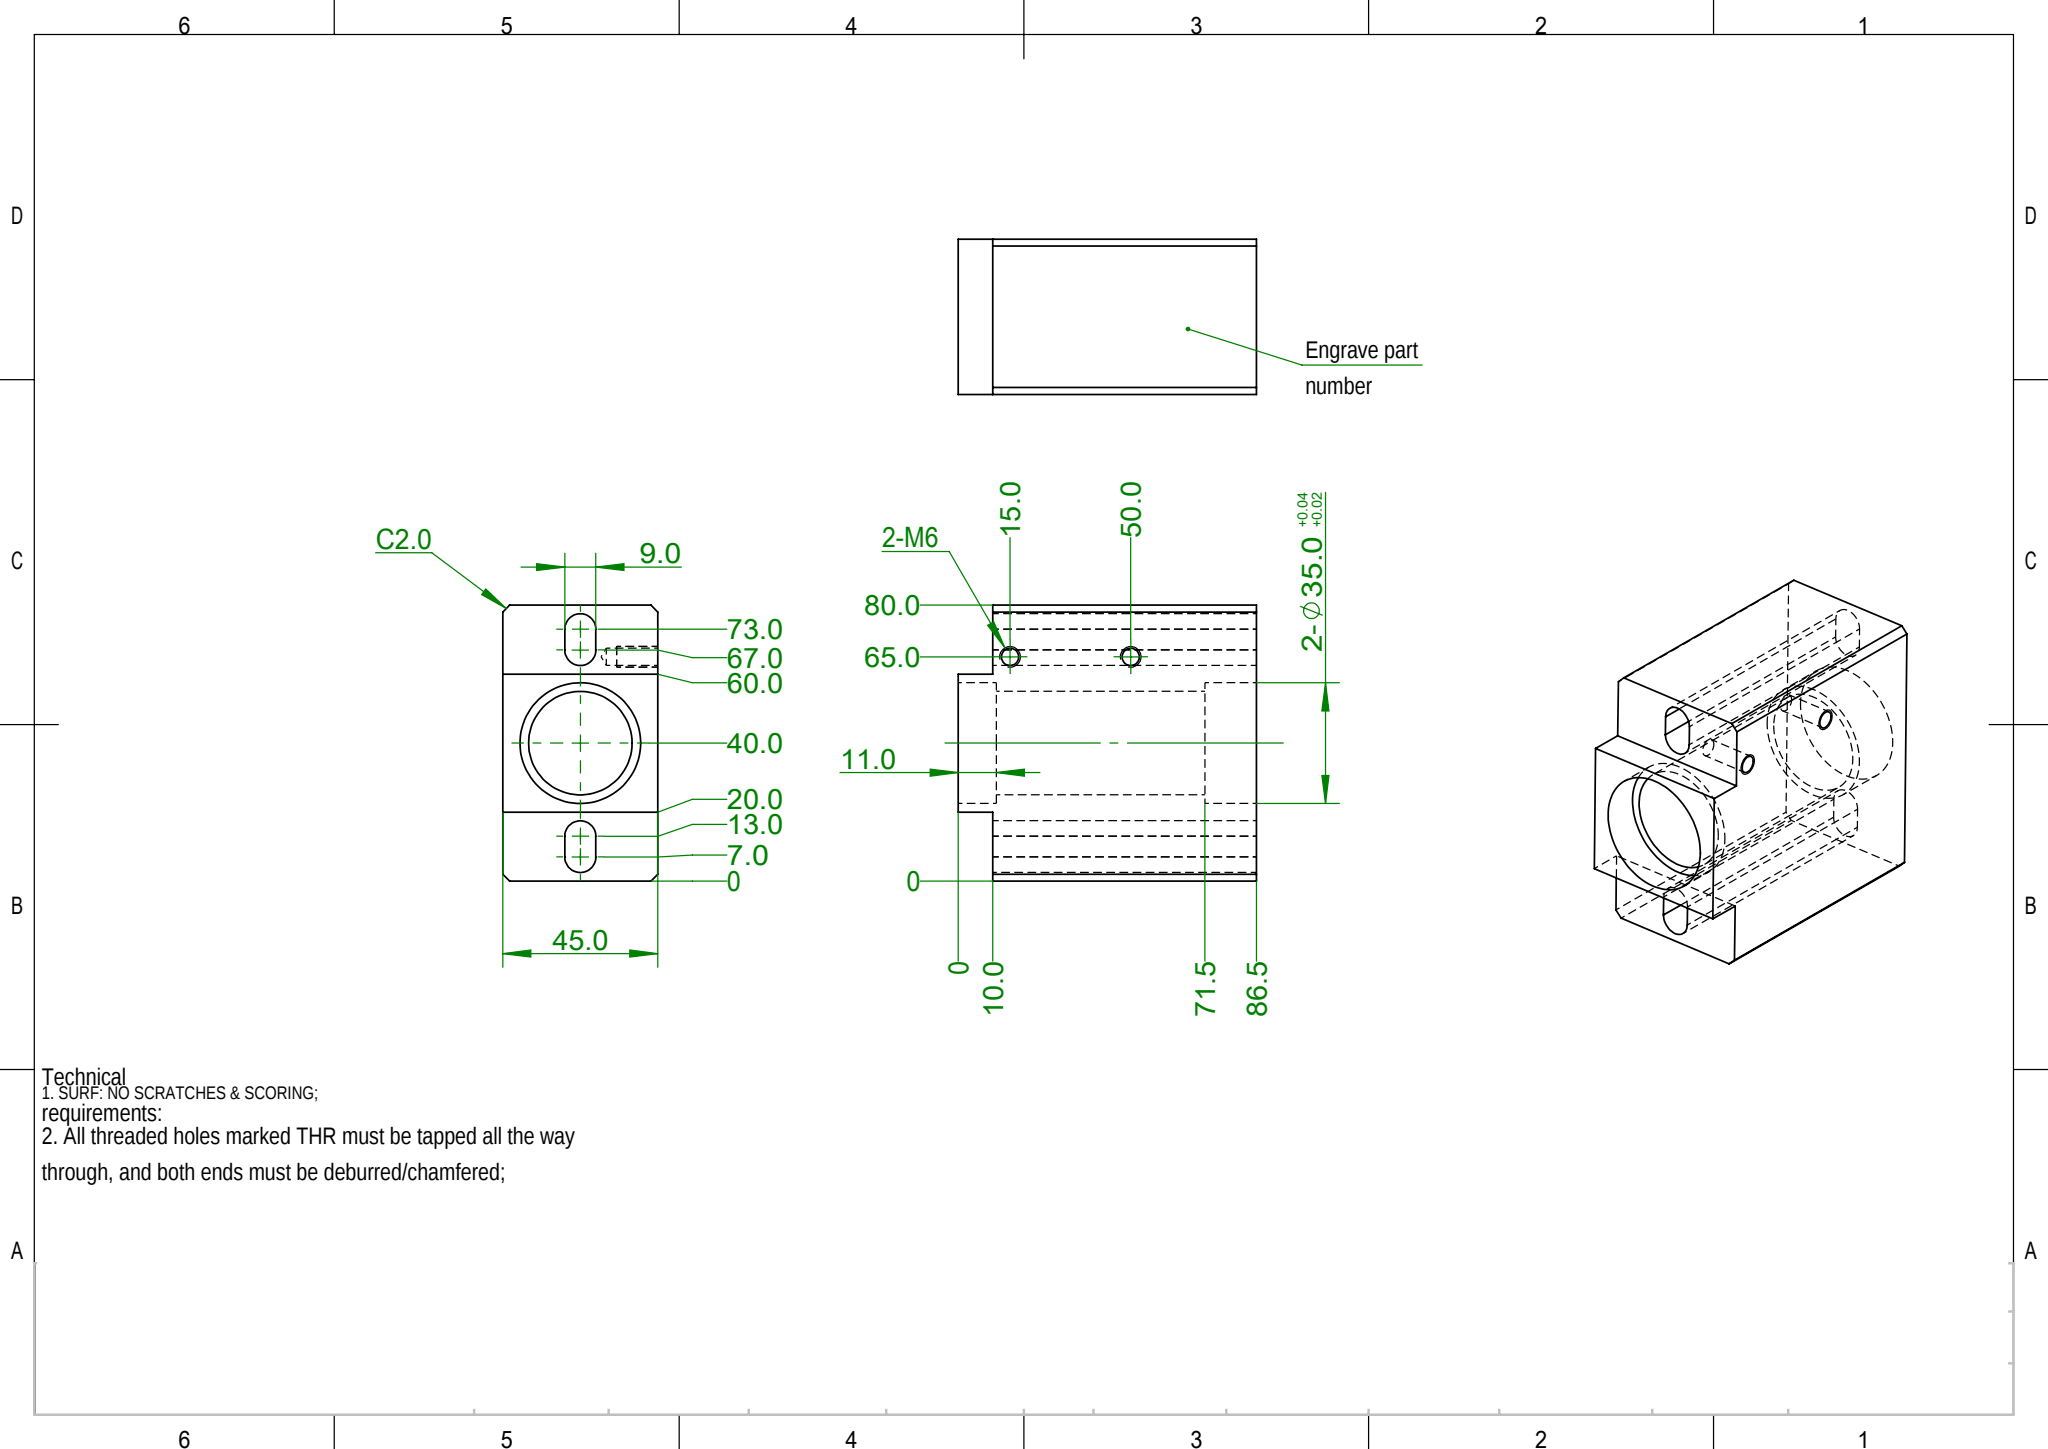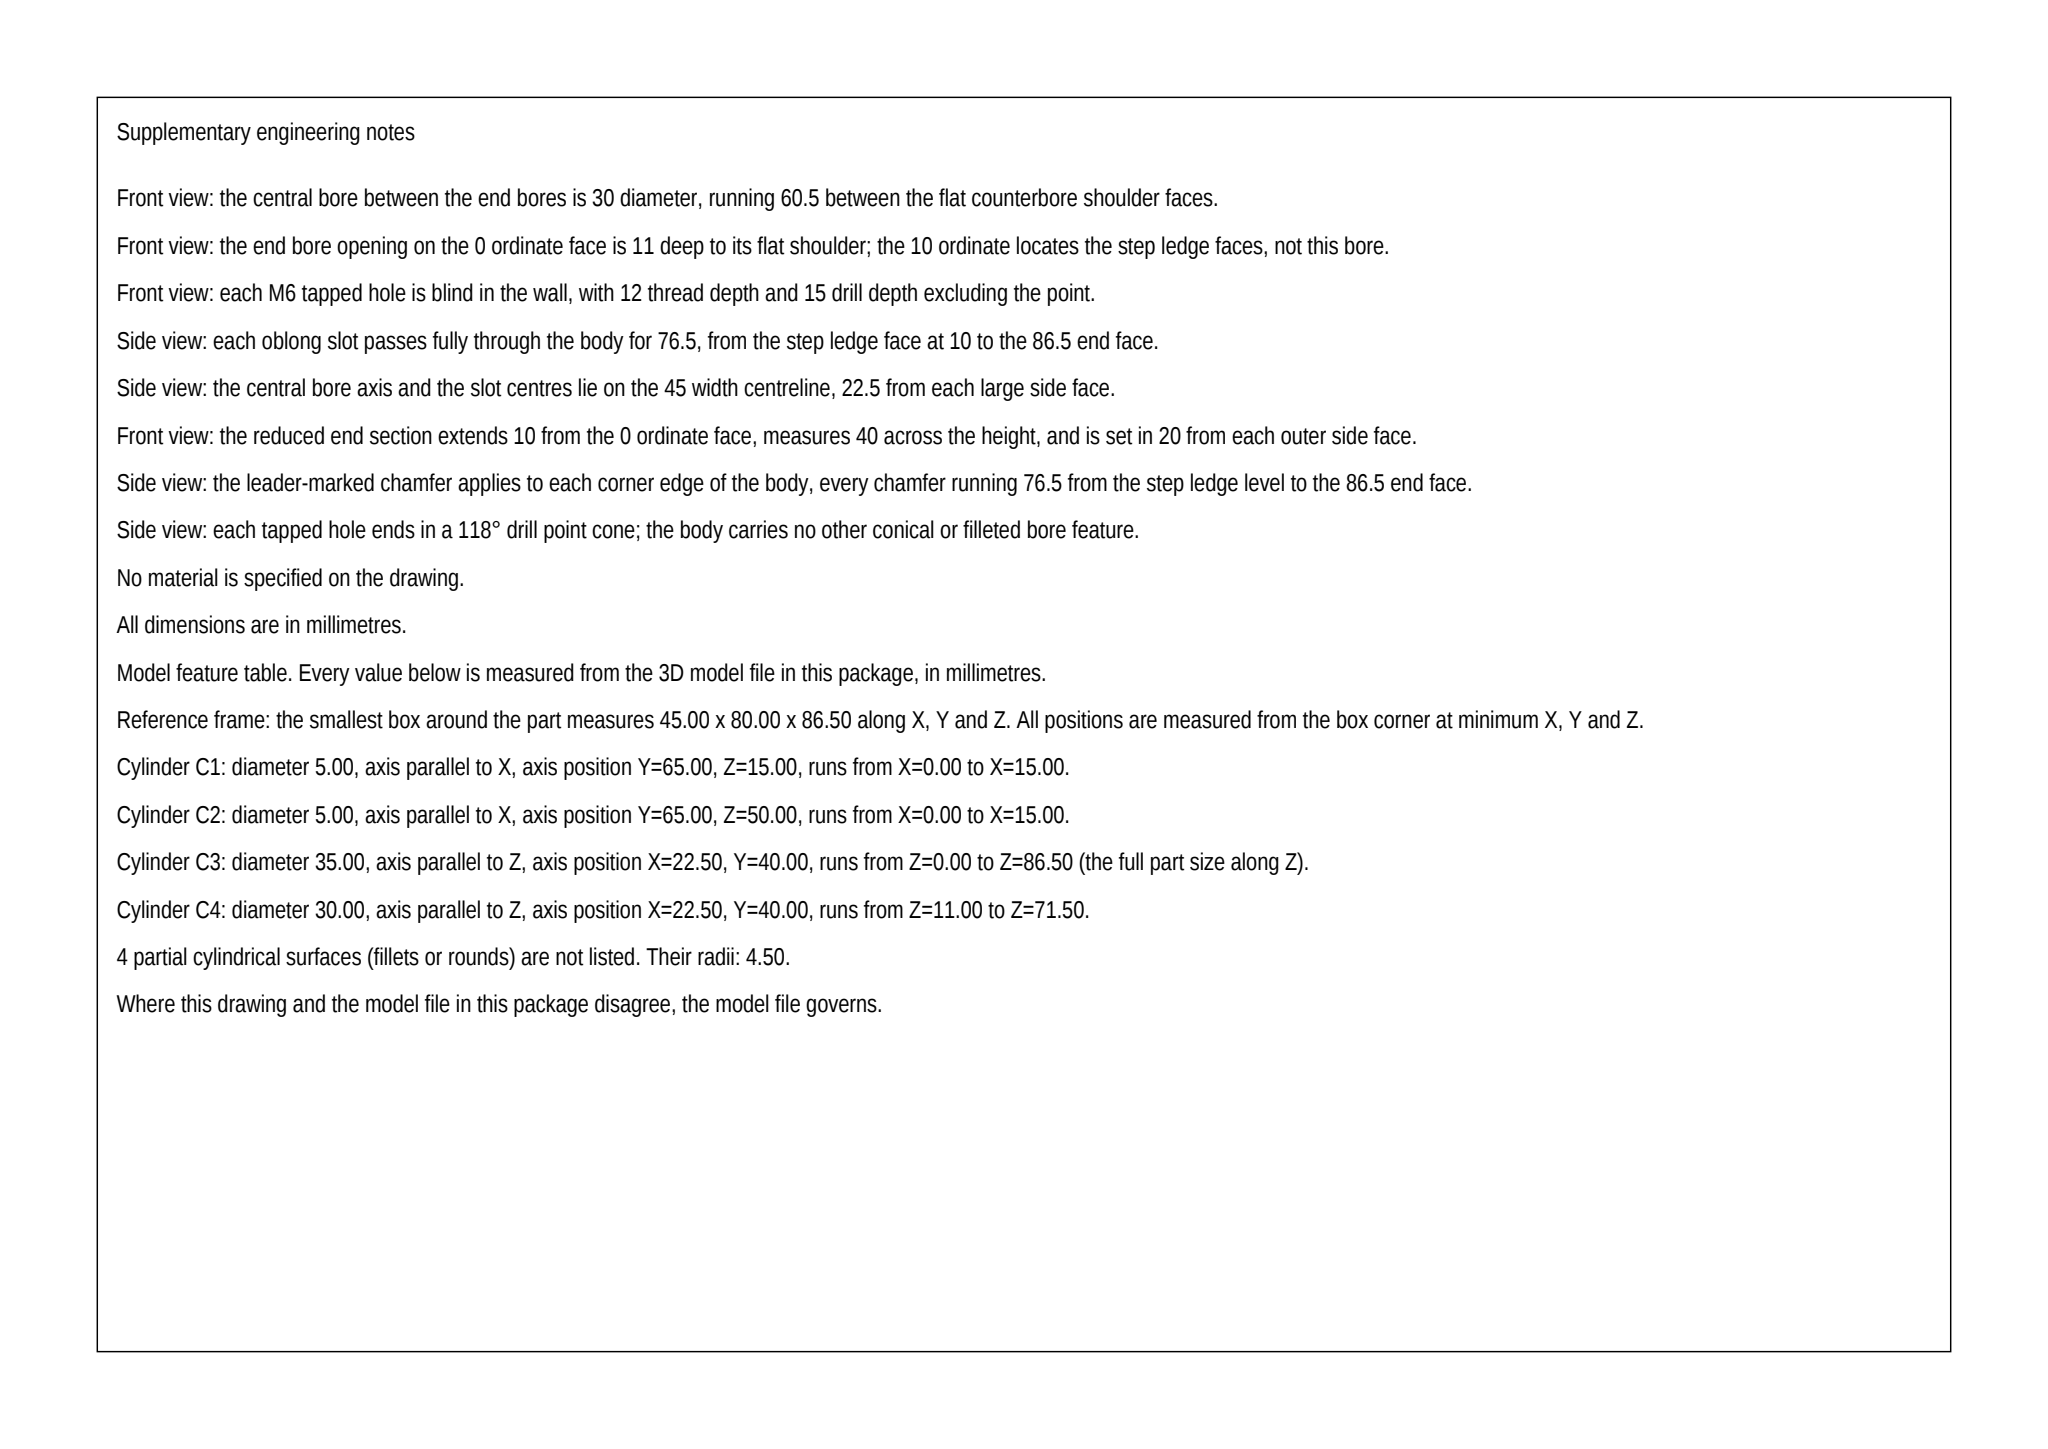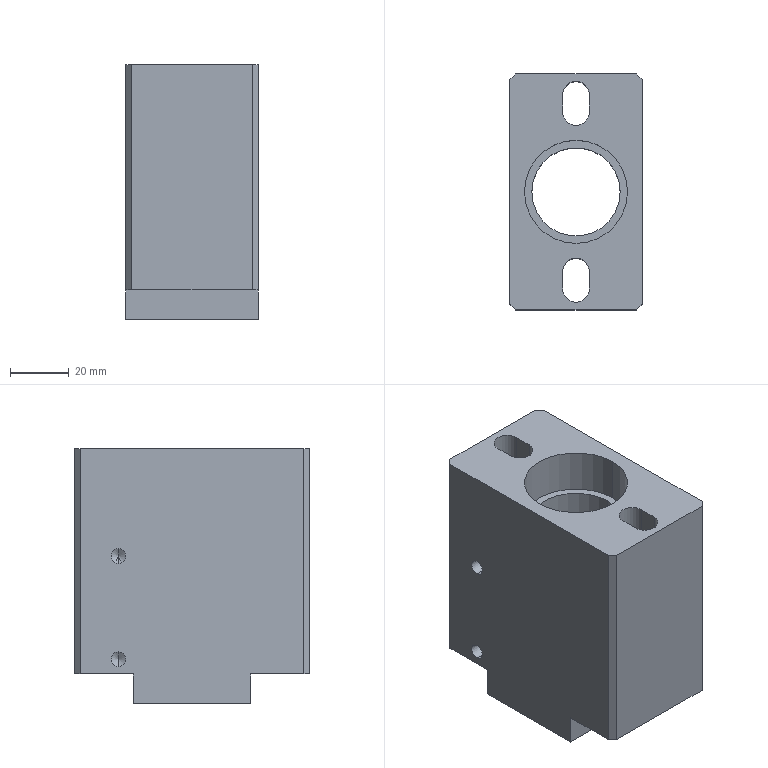Part | SolidWorks | mm | 1 solid | 38 faces | box 45 x 80 x 86.5 mm | volume 206404 mm3 | plane 20 | cylinder 14 | cone 4 | commonest cylinder face diameters 5 x4 35 x4 9 x4 30 x2
Drawing notes:
Ø30 THRU BORE BTWN 2-Ø35 C'BORES | from the solid: cyl dia 30 axis z at (22.5,40) len 60.5 between Ø35 c'bores 11 & 15 deep; 11+60.5+15=86.5 total
2-M6 DP 15 FROM NEAR FACE SHOWN IN FRONT VIEW | from the solid: 2 x Ø5 cyls axis x, len 15, at y65/z15 and y65/z50, 118° drill point; block x extent 0-45
build123d program:
from build123d import *

# Parameters (mm, degrees)
SKETCH1_W             = 45
SKETCH1_H             = 80
BOSS_EXTRUDE1_DEPTH   = 86.5
SKETCH2_R             = 15
CUT_EXTRUDE1_DEPTH    = 555.5
SKETCH4_R             = 17.5
CUT_EXTRUDE2_DEPTH    = 15
CUT_EXTRUDE3_START    = -11
SKETCH5_R             = 17.5
CUT_EXTRUDE3_DEPTH    = 11
M6_TAPPED_HOLE1_D     = 5
M6_TAPPED_HOLE1_DEPTH = 15
M6_TAPPED_HOLE1_TIP   = 1.502
CHAMFER2_SIZE         = 2
CUT_EXTRUDE4_DEPTH    = 111
SKETCH9_W             = 104.782
SKETCH9_H             = 36.571
CUT_EXTRUDE5_DEPTH    = 10


with BuildPart() as part:
    # Sketch1 → Boss-Extrude1 (new body)
    with BuildSketch(Plane.XY):
        Rectangle(SKETCH1_W, SKETCH1_H)
    extrude(amount=BOSS_EXTRUDE1_DEPTH)

    # Sketch2 → Cut-Extrude1 (cut, symmetric)
    with BuildSketch(Plane.XY):
        with Locations(Location((0, 0, 0), (0, 0, 180))):
            Circle(SKETCH2_R)
    extrude(amount=CUT_EXTRUDE1_DEPTH, both=True, mode=Mode.SUBTRACT)

    # Sketch4 → Cut-Extrude2 (cut)
    with BuildSketch(Plane.XY.offset(86.5)):
        Circle(SKETCH4_R)
    extrude(amount=-CUT_EXTRUDE2_DEPTH, mode=Mode.SUBTRACT)

    # Sketch5 → Cut-Extrude3 (cut)
    with BuildSketch(Plane(origin=(0, 0, 0), x_dir=(-1, 0, 0), z_dir=(0, 0, -1)).offset(CUT_EXTRUDE3_START)):
        with Locations(Location((0, 0, 0), (0, 0, 180))):
            Circle(SKETCH5_R)
    extrude(amount=CUT_EXTRUDE3_DEPTH, mode=Mode.SUBTRACT)

    # M6 Tapped Hole1
    with Locations(Plane.ZY.offset(22.5)):
        with Locations((15, 25), (50, 25)):
            Hole(M6_TAPPED_HOLE1_D / 2, depth=M6_TAPPED_HOLE1_DEPTH)
            with Locations((0, 0, -(M6_TAPPED_HOLE1_DEPTH + M6_TAPPED_HOLE1_TIP / 2))):  # 118° drill point
                Cone(0, M6_TAPPED_HOLE1_D / 2, M6_TAPPED_HOLE1_TIP, mode=Mode.SUBTRACT)

    # Chamfer2
    chamfer2_edges = [part.edges().sort_by_distance(p)[0] for p in [
        (-22.5, 40, 43.25),
        (22.5, 40, 43.25),
        (22.5, -40, 43.25),
        (-22.5, -40, 43.25),
    ]]
    chamfer(chamfer2_edges, length=CHAMFER2_SIZE)

    # Sketch8 → Cut-Extrude4 (cut)
    with BuildSketch(Plane(origin=(0, 0, 0), x_dir=(-1, 0, 0), z_dir=(0, 0, -1))):
        with BuildLine():
            Line((4.5, 33), (4.5, 27))
            ThreePointArc((4.5, 27), (0, 22.5), (-4.5, 27))
            Line((-4.5, 27), (-4.5, 33))
            ThreePointArc((-4.5, 33), (0, 37.5), (4.5, 33))
        make_face()
        with BuildLine():
            Line((-4.5, -33), (-4.5, -27))
            ThreePointArc((-4.5, -27), (0, -22.5), (4.5, -27))
            Line((4.5, -27), (4.5, -33))
            ThreePointArc((4.5, -33), (0, -37.5), (-4.5, -33))
        make_face()
    extrude(amount=-CUT_EXTRUDE4_DEPTH, mode=Mode.SUBTRACT)

    # Sketch9 → Cut-Extrude5 (cut)
    with BuildSketch(Plane(origin=(0, 0, 0), x_dir=(-1, 0, 0), z_dir=(0, 0, -1))):
        with Locations((1.592, 38.285)):
            Rectangle(SKETCH9_W, SKETCH9_H)
        with Locations((1.592, -38.285)):
            Rectangle(SKETCH9_W, SKETCH9_H)
    extrude(amount=-CUT_EXTRUDE5_DEPTH, mode=Mode.SUBTRACT)


solid = part.part